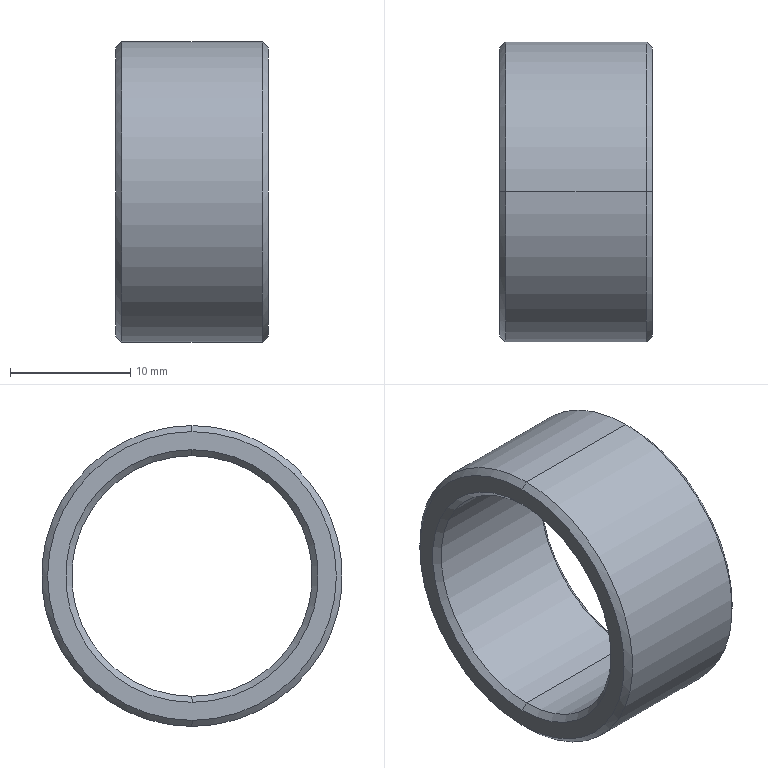Component | SolidWorks | ChainPartDrivenShaftLocatingSleeve-1 | 1 solid | 14 faces | box 12.7 x 25 x 25 mm | volume 2209 mm3 | cone 8 | cylinder 4 | plane 2 | commonest cylinder face diameters 20 x2 25 x2
build123d program:
from build123d import *

# Parameters (mm, degrees)
SKETCH1_R           = 12.5
SKETCH1_R_2         = 10
BOSS_EXTRUDE1_DEPTH = 6.35
CHAMFER1_SIZE       = 0.5


with BuildPart() as part:
    # Sketch1 → Boss-Extrude1 (new, symmetric)
    with BuildSketch(Plane.XY):
        Circle(SKETCH1_R)
        Circle(SKETCH1_R_2, mode=Mode.SUBTRACT)
    extrude(amount=BOSS_EXTRUDE1_DEPTH, both=True)

    # Chamfer1
    chamfer1_edges = [part.edges().sort_by_distance(p)[0] for p in [
        (-12.5, 0, -6.35),
        (-12.5, 0, 6.35),
        (-10, 0, -6.35),
        (-10, 0, 6.35),
    ]]
    chamfer(chamfer1_edges, length=CHAMFER1_SIZE)


solid = part.part

# Placed as in the assembly
solid = solid.moved(Location((94.587, -2.563, -673.885), (0, 90, 0)))